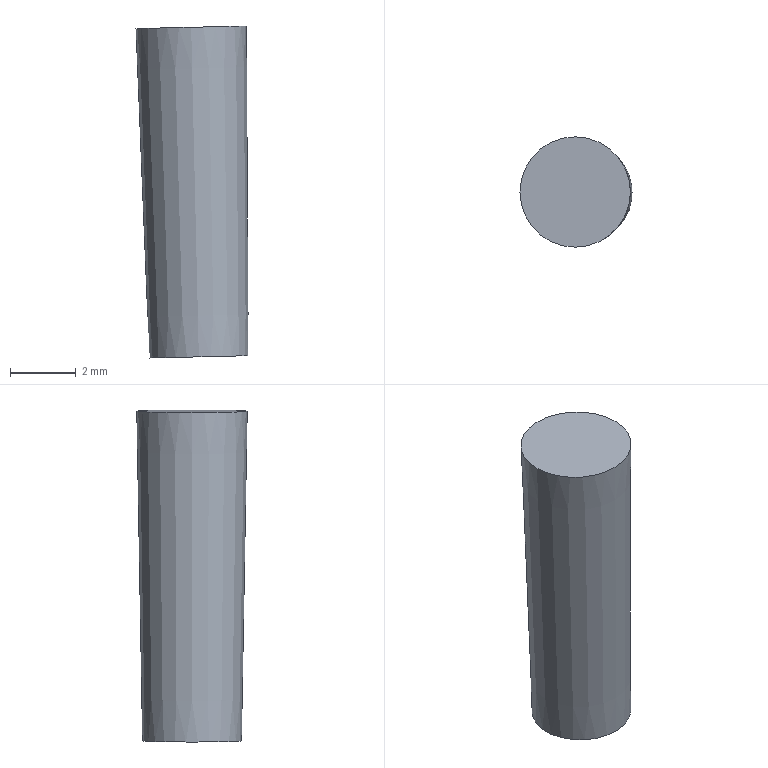Component | NX | PIN | 1 solid | 3 faces | box 3.41 x 3.35 x 10.07 mm | volume 79 mm3 | plane 2 | cone 1
STEP:
#1=CARTESIAN_POINT('',(0.,0.,0.));
#2=DIRECTION('',(0.,0.,1.));
#3=DIRECTION('',(1.,0.,0.));
#4=AXIS2_PLACEMENT_3D('',#1,#2,#3);
#5=CARTESIAN_POINT('',(-32.398,-12.5,108.101));
#6=VERTEX_POINT('',#5);
#7=CARTESIAN_POINT('',(-32.398,-11.,108.101));
#8=DIRECTION('',(-0.02318,0.,0.9997));
#9=DIRECTION('',(0.,-1.,0.));
#10=AXIS2_PLACEMENT_3D('',#7,#8,#9);
#11=CIRCLE('',#10,1.5);
#12=CARTESIAN_POINT('',(-32.398,-12.5,108.101));
#13=DIRECTION('',(0.02318,0.,-0.9997));
#14=DIRECTION('',(0.,1.,0.));
#15=AXIS2_PLACEMENT_3D('',#12,#13,#14);
#16=PLANE('',#15);
#17=CARTESIAN_POINT('',(0.,0.));
#18=CARTESIAN_POINT('',(0.,2.598));
#19=CARTESIAN_POINT('',(2.25,1.299));
#20=CARTESIAN_POINT('',(4.5,0.));
#21=CARTESIAN_POINT('',(2.25,-1.299));
#22=CARTESIAN_POINT('',(0.,-2.598));
#23=CARTESIAN_POINT('',(0.,0.));
#24=(BOUNDED_CURVE()B_SPLINE_CURVE(2,(#17,#18,#19,#20,#21,#22,#23),.UNSPECIFIED.,.T.,.F.)B_SPLINE_CURVE_WITH_KNOTS((1,2,2,2,2,1),(-2.094,0.,2.094,4.189,6.283,8.378),.UNSPECIFIED.)CURVE()GEOMETRIC_REPRESENTATION_ITEM()RATIONAL_B_SPLINE_CURVE((1.,0.5,1.,0.5,1.,0.5,1.))REPRESENTATION_ITEM(''));
#25=(GEOMETRIC_REPRESENTATION_CONTEXT(2)PARAMETRIC_REPRESENTATION_CONTEXT()REPRESENTATION_CONTEXT('',''));
#26=DEFINITIONAL_REPRESENTATION('',(#24),#25);
#27=PCURVE('',#16,#26);
#28=CARTESIAN_POINT('',(-32.63,-11.,118.098));
#29=DIRECTION('',(-0.02318,0.,0.9997));
#30=DIRECTION('',(-0.,-1.,-0.));
#31=AXIS2_PLACEMENT_3D('',#28,#29,#30);
#32=CONICAL_SURFACE('',#31,1.675,0.01745);
#33=CARTESIAN_POINT('',(0.,-10.));
#34=DIRECTION('',(1.,0.));
#35=VECTOR('',#34,1.);
#36=LINE('',#33,#35);
#37=(GEOMETRIC_REPRESENTATION_CONTEXT(2)PARAMETRIC_REPRESENTATION_CONTEXT()REPRESENTATION_CONTEXT('',''));
#38=DEFINITIONAL_REPRESENTATION('',(#36),#37);
#39=PCURVE('',#32,#38);
#40=SURFACE_CURVE('',#11,(#27,#39),.PCURVE_S1.);
#41=EDGE_CURVE('',#6,#6,#40,.T.);
#42=ORIENTED_EDGE('',*,*,#41,.F.);
#43=EDGE_LOOP('',(#42));
#44=FACE_BOUND('',#43,.T.);
#45=ADVANCED_FACE('',(#44),#16,.T.);
#46=ORIENTED_EDGE('',*,*,#41,.T.);
#47=CARTESIAN_POINT('',(-32.63,-12.675,118.098));
#48=VERTEX_POINT('',#47);
#49=CARTESIAN_POINT('',(-32.398,-12.5,108.101));
#50=CARTESIAN_POINT('',(-32.63,-12.675,118.098));
#51=B_SPLINE_CURVE_WITH_KNOTS('',1,(#49,#50),.UNSPECIFIED.,.F.,.F.,(2,2),(-10.002,0.),.PIECEWISE_BEZIER_KNOTS.);
#52=CARTESIAN_POINT('',(6.283,0.));
#53=DIRECTION('',(0.,1.));
#54=VECTOR('',#53,1.);
#55=LINE('',#52,#54);
#56=(GEOMETRIC_REPRESENTATION_CONTEXT(2)PARAMETRIC_REPRESENTATION_CONTEXT()REPRESENTATION_CONTEXT('',''));
#57=DEFINITIONAL_REPRESENTATION('',(#55),#56);
#58=PCURVE('',#32,#57);
#59=CARTESIAN_POINT('',(0.,0.));
#60=DIRECTION('',(0.,1.));
#61=VECTOR('',#60,1.);
#62=LINE('',#59,#61);
#63=(GEOMETRIC_REPRESENTATION_CONTEXT(2)PARAMETRIC_REPRESENTATION_CONTEXT()REPRESENTATION_CONTEXT('',''));
#64=DEFINITIONAL_REPRESENTATION('',(#62),#63);
#65=PCURVE('',#32,#64);
#66=SEAM_CURVE('',#51,(#58,#65),.PCURVE_S1.);
#67=EDGE_CURVE('',#6,#48,#66,.T.);
#68=ORIENTED_EDGE('',*,*,#67,.T.);
#69=CARTESIAN_POINT('',(-32.63,-11.,118.098));
#70=DIRECTION('',(-0.02318,0.,0.9997));
#71=DIRECTION('',(0.,-1.,0.));
#72=AXIS2_PLACEMENT_3D('',#69,#70,#71);
#73=CIRCLE('',#72,1.675);
#74=CARTESIAN_POINT('',(0.,0.));
#75=DIRECTION('',(1.,0.));
#76=VECTOR('',#75,1.);
#77=LINE('',#74,#76);
#78=(GEOMETRIC_REPRESENTATION_CONTEXT(2)PARAMETRIC_REPRESENTATION_CONTEXT()REPRESENTATION_CONTEXT('',''));
#79=DEFINITIONAL_REPRESENTATION('',(#77),#78);
#80=PCURVE('',#32,#79);
#81=CARTESIAN_POINT('',(-32.63,-11.,118.098));
#82=DIRECTION('',(-0.02318,0.,0.9997));
#83=DIRECTION('',(0.,-1.,0.));
#84=AXIS2_PLACEMENT_3D('',#81,#82,#83);
#85=PLANE('',#84);
#86=CARTESIAN_POINT('',(0.,0.));
#87=DIRECTION('',(1.,0.));
#88=AXIS2_PLACEMENT_2D('',#86,#87);
#89=CIRCLE('',#88,1.675);
#90=(GEOMETRIC_REPRESENTATION_CONTEXT(2)PARAMETRIC_REPRESENTATION_CONTEXT()REPRESENTATION_CONTEXT('',''));
#91=DEFINITIONAL_REPRESENTATION('',(#89),#90);
#92=PCURVE('',#85,#91);
#93=SURFACE_CURVE('',#73,(#80,#92),.PCURVE_S1.);
#94=EDGE_CURVE('',#48,#48,#93,.T.);
#95=ORIENTED_EDGE('',*,*,#94,.F.);
#96=ORIENTED_EDGE('',*,*,#67,.F.);
#97=EDGE_LOOP('',(#46,#68,#95,#96));
#98=FACE_BOUND('',#97,.T.);
#99=ADVANCED_FACE('',(#98),#32,.T.);
#100=ORIENTED_EDGE('',*,*,#94,.T.);
#101=EDGE_LOOP('',(#100));
#102=FACE_BOUND('',#101,.T.);
#103=ADVANCED_FACE('',(#102),#85,.T.);
#104=CLOSED_SHELL('',(#45,#99,#103));
#105=MANIFOLD_SOLID_BREP('',#104);
#106=(LENGTH_UNIT()NAMED_UNIT(*)SI_UNIT(.MILLI.,.METRE.));
#107=UNCERTAINTY_MEASURE_WITH_UNIT(LENGTH_MEASURE(0.00001),#106,'','');
#108=(NAMED_UNIT(*)PLANE_ANGLE_UNIT()SI_UNIT($,.RADIAN.));
#109=(NAMED_UNIT(*)SI_UNIT($,.STERADIAN.)SOLID_ANGLE_UNIT());
#110=(GEOMETRIC_REPRESENTATION_CONTEXT(3)GLOBAL_UNCERTAINTY_ASSIGNED_CONTEXT((#107))GLOBAL_UNIT_ASSIGNED_CONTEXT((#106,#108,#109))REPRESENTATION_CONTEXT('',''));
#111=ADVANCED_BREP_SHAPE_REPRESENTATION('',(#4,#105),#110);